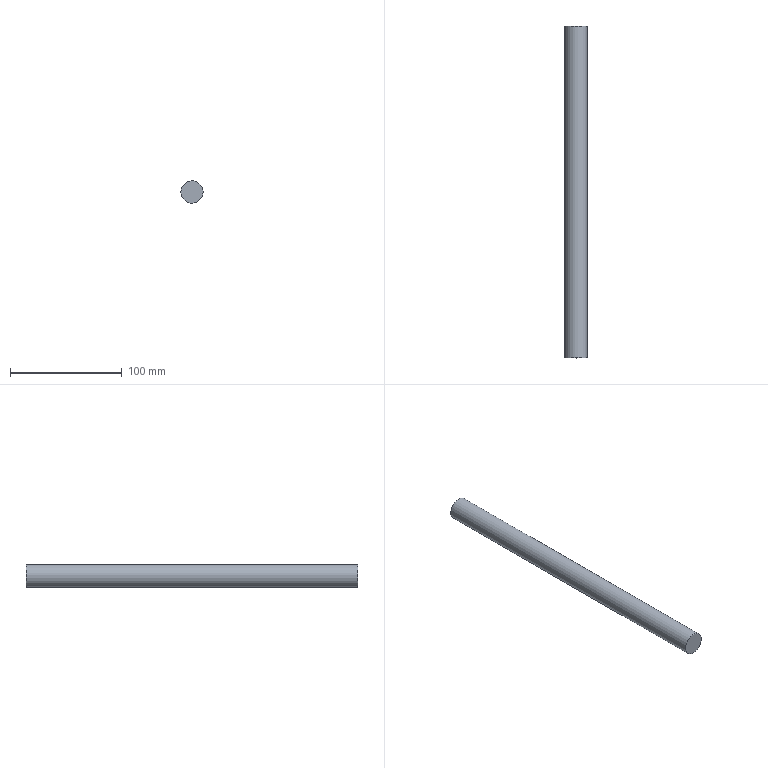Component | NX | 131_SHAFT_2 | 1 solid | 3 faces | box 20 x 297 x 20 mm | volume 93305 mm3 | plane 2 | cylinder 1 | commonest cylinder face diameters 20 x1
STEP:
#1=CARTESIAN_POINT('',(0.,0.,0.));
#2=DIRECTION('',(0.,0.,1.));
#3=DIRECTION('',(1.,0.,0.));
#4=AXIS2_PLACEMENT_3D('',#1,#2,#3);
#5=CARTESIAN_POINT('',(609.988,-154.,-0.4959));
#6=VERTEX_POINT('',#5);
#7=CARTESIAN_POINT('',(600.,-154.,-0.));
#8=DIRECTION('',(-0.,-1.,-0.));
#9=DIRECTION('',(0.9988,-0.,-0.04959));
#10=AXIS2_PLACEMENT_3D('',#7,#8,#9);
#11=CIRCLE('',#10,10.);
#12=CARTESIAN_POINT('',(600.,-154.,-0.));
#13=DIRECTION('',(0.,1.,0.));
#14=DIRECTION('',(0.04959,-0.,0.9988));
#15=AXIS2_PLACEMENT_3D('',#12,#13,#14);
#16=CYLINDRICAL_SURFACE('',#15,10.);
#17=CARTESIAN_POINT('',(7.854,0.));
#18=DIRECTION('',(-1.,0.));
#19=VECTOR('',#18,1.);
#20=LINE('',#17,#19);
#21=(GEOMETRIC_REPRESENTATION_CONTEXT(2)PARAMETRIC_REPRESENTATION_CONTEXT()REPRESENTATION_CONTEXT('',''));
#22=DEFINITIONAL_REPRESENTATION('',(#20),#21);
#23=PCURVE('',#16,#22);
#24=CARTESIAN_POINT('',(600.,-154.,-0.));
#25=DIRECTION('',(-0.,-1.,-0.));
#26=DIRECTION('',(-0.04959,0.,-0.9988));
#27=AXIS2_PLACEMENT_3D('',#24,#25,#26);
#28=PLANE('',#27);
#29=CARTESIAN_POINT('',(0.,0.));
#30=DIRECTION('',(-0.,1.));
#31=AXIS2_PLACEMENT_2D('',#29,#30);
#32=CIRCLE('',#31,10.);
#33=(GEOMETRIC_REPRESENTATION_CONTEXT(2)PARAMETRIC_REPRESENTATION_CONTEXT()REPRESENTATION_CONTEXT('',''));
#34=DEFINITIONAL_REPRESENTATION('',(#32),#33);
#35=PCURVE('',#28,#34);
#36=SURFACE_CURVE('',#11,(#23,#35),.PCURVE_S1.);
#37=EDGE_CURVE('',#6,#6,#36,.T.);
#38=ORIENTED_EDGE('',*,*,#37,.F.);
#39=CARTESIAN_POINT('',(609.988,143.,-0.4959));
#40=VERTEX_POINT('',#39);
#41=CARTESIAN_POINT('',(609.988,-154.,-0.4959));
#42=CARTESIAN_POINT('',(609.988,143.,-0.4959));
#43=B_SPLINE_CURVE_WITH_KNOTS('',1,(#41,#42),.UNSPECIFIED.,.F.,.F.,(2,2),(0.,297.),.PIECEWISE_BEZIER_KNOTS.);
#44=CARTESIAN_POINT('',(7.854,0.));
#45=DIRECTION('',(0.,1.));
#46=VECTOR('',#45,1.);
#47=LINE('',#44,#46);
#48=(GEOMETRIC_REPRESENTATION_CONTEXT(2)PARAMETRIC_REPRESENTATION_CONTEXT()REPRESENTATION_CONTEXT('',''));
#49=DEFINITIONAL_REPRESENTATION('',(#47),#48);
#50=PCURVE('',#16,#49);
#51=CARTESIAN_POINT('',(1.571,0.));
#52=DIRECTION('',(0.,1.));
#53=VECTOR('',#52,1.);
#54=LINE('',#51,#53);
#55=(GEOMETRIC_REPRESENTATION_CONTEXT(2)PARAMETRIC_REPRESENTATION_CONTEXT()REPRESENTATION_CONTEXT('',''));
#56=DEFINITIONAL_REPRESENTATION('',(#54),#55);
#57=PCURVE('',#16,#56);
#58=SEAM_CURVE('',#43,(#50,#57),.PCURVE_S1.);
#59=EDGE_CURVE('',#6,#40,#58,.T.);
#60=ORIENTED_EDGE('',*,*,#59,.T.);
#61=CARTESIAN_POINT('',(600.,143.,-0.));
#62=DIRECTION('',(0.,1.,0.));
#63=DIRECTION('',(0.9988,-0.,-0.04959));
#64=AXIS2_PLACEMENT_3D('',#61,#62,#63);
#65=CIRCLE('',#64,10.);
#66=CARTESIAN_POINT('',(1.571,297.));
#67=DIRECTION('',(1.,0.));
#68=VECTOR('',#67,1.);
#69=LINE('',#66,#68);
#70=(GEOMETRIC_REPRESENTATION_CONTEXT(2)PARAMETRIC_REPRESENTATION_CONTEXT()REPRESENTATION_CONTEXT('',''));
#71=DEFINITIONAL_REPRESENTATION('',(#69),#70);
#72=PCURVE('',#16,#71);
#73=CARTESIAN_POINT('',(600.,143.,-0.));
#74=DIRECTION('',(0.,1.,0.));
#75=DIRECTION('',(0.04959,-0.,0.9988));
#76=AXIS2_PLACEMENT_3D('',#73,#74,#75);
#77=PLANE('',#76);
#78=CARTESIAN_POINT('',(0.,0.));
#79=DIRECTION('',(0.,1.));
#80=AXIS2_PLACEMENT_2D('',#78,#79);
#81=CIRCLE('',#80,10.);
#82=(GEOMETRIC_REPRESENTATION_CONTEXT(2)PARAMETRIC_REPRESENTATION_CONTEXT()REPRESENTATION_CONTEXT('',''));
#83=DEFINITIONAL_REPRESENTATION('',(#81),#82);
#84=PCURVE('',#77,#83);
#85=SURFACE_CURVE('',#65,(#72,#84),.PCURVE_S1.);
#86=EDGE_CURVE('',#40,#40,#85,.T.);
#87=ORIENTED_EDGE('',*,*,#86,.F.);
#88=ORIENTED_EDGE('',*,*,#59,.F.);
#89=EDGE_LOOP('',(#38,#60,#87,#88));
#90=FACE_BOUND('',#89,.T.);
#91=ADVANCED_FACE('',(#90),#16,.T.);
#92=ORIENTED_EDGE('',*,*,#37,.T.);
#93=EDGE_LOOP('',(#92));
#94=FACE_BOUND('',#93,.T.);
#95=ADVANCED_FACE('',(#94),#28,.T.);
#96=ORIENTED_EDGE('',*,*,#86,.T.);
#97=EDGE_LOOP('',(#96));
#98=FACE_BOUND('',#97,.T.);
#99=ADVANCED_FACE('',(#98),#77,.T.);
#100=CLOSED_SHELL('',(#91,#95,#99));
#101=MANIFOLD_SOLID_BREP('',#100);
#102=(LENGTH_UNIT()NAMED_UNIT(*)SI_UNIT(.MILLI.,.METRE.));
#103=UNCERTAINTY_MEASURE_WITH_UNIT(LENGTH_MEASURE(0.00001),#102,'','');
#104=(NAMED_UNIT(*)PLANE_ANGLE_UNIT()SI_UNIT($,.RADIAN.));
#105=(NAMED_UNIT(*)SI_UNIT($,.STERADIAN.)SOLID_ANGLE_UNIT());
#106=(GEOMETRIC_REPRESENTATION_CONTEXT(3)GLOBAL_UNCERTAINTY_ASSIGNED_CONTEXT((#103))GLOBAL_UNIT_ASSIGNED_CONTEXT((#102,#104,#105))REPRESENTATION_CONTEXT('',''));
#107=ADVANCED_BREP_SHAPE_REPRESENTATION('',(#4,#101),#106);